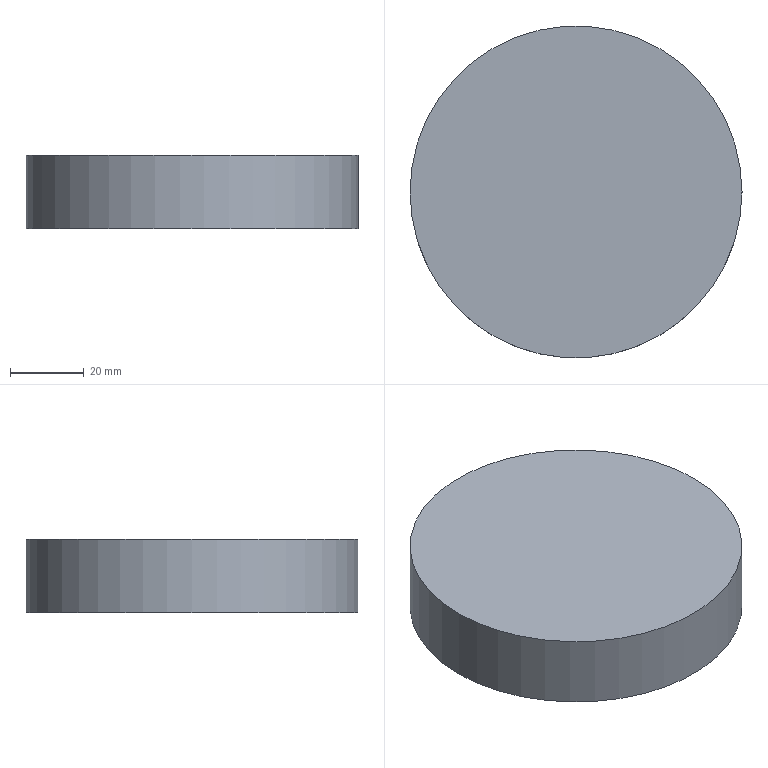CAM job | NX | mm | 3-axis | 1 set-up | 2 operations | part box 90 x 90 x 20
set-up 1
1. Cavity Milling | Mill Mill5 20 | CAVITY_MILL | path 306861.397 mm | 123.526 min
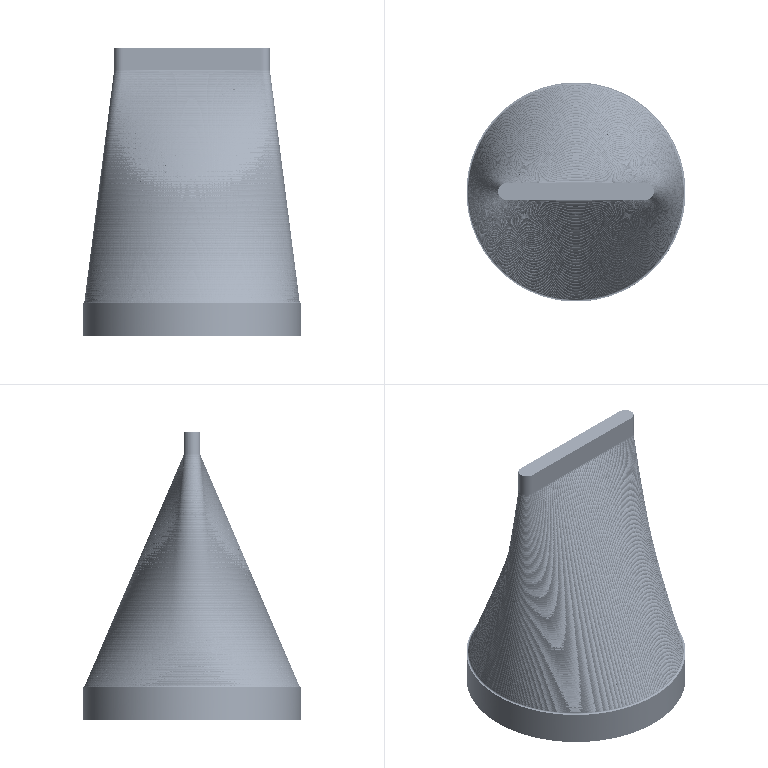2. Z-Level Milling | Mill Mill5 20 | ZLEVEL_PROFILE | path 132990.39 mm | 53.146 min